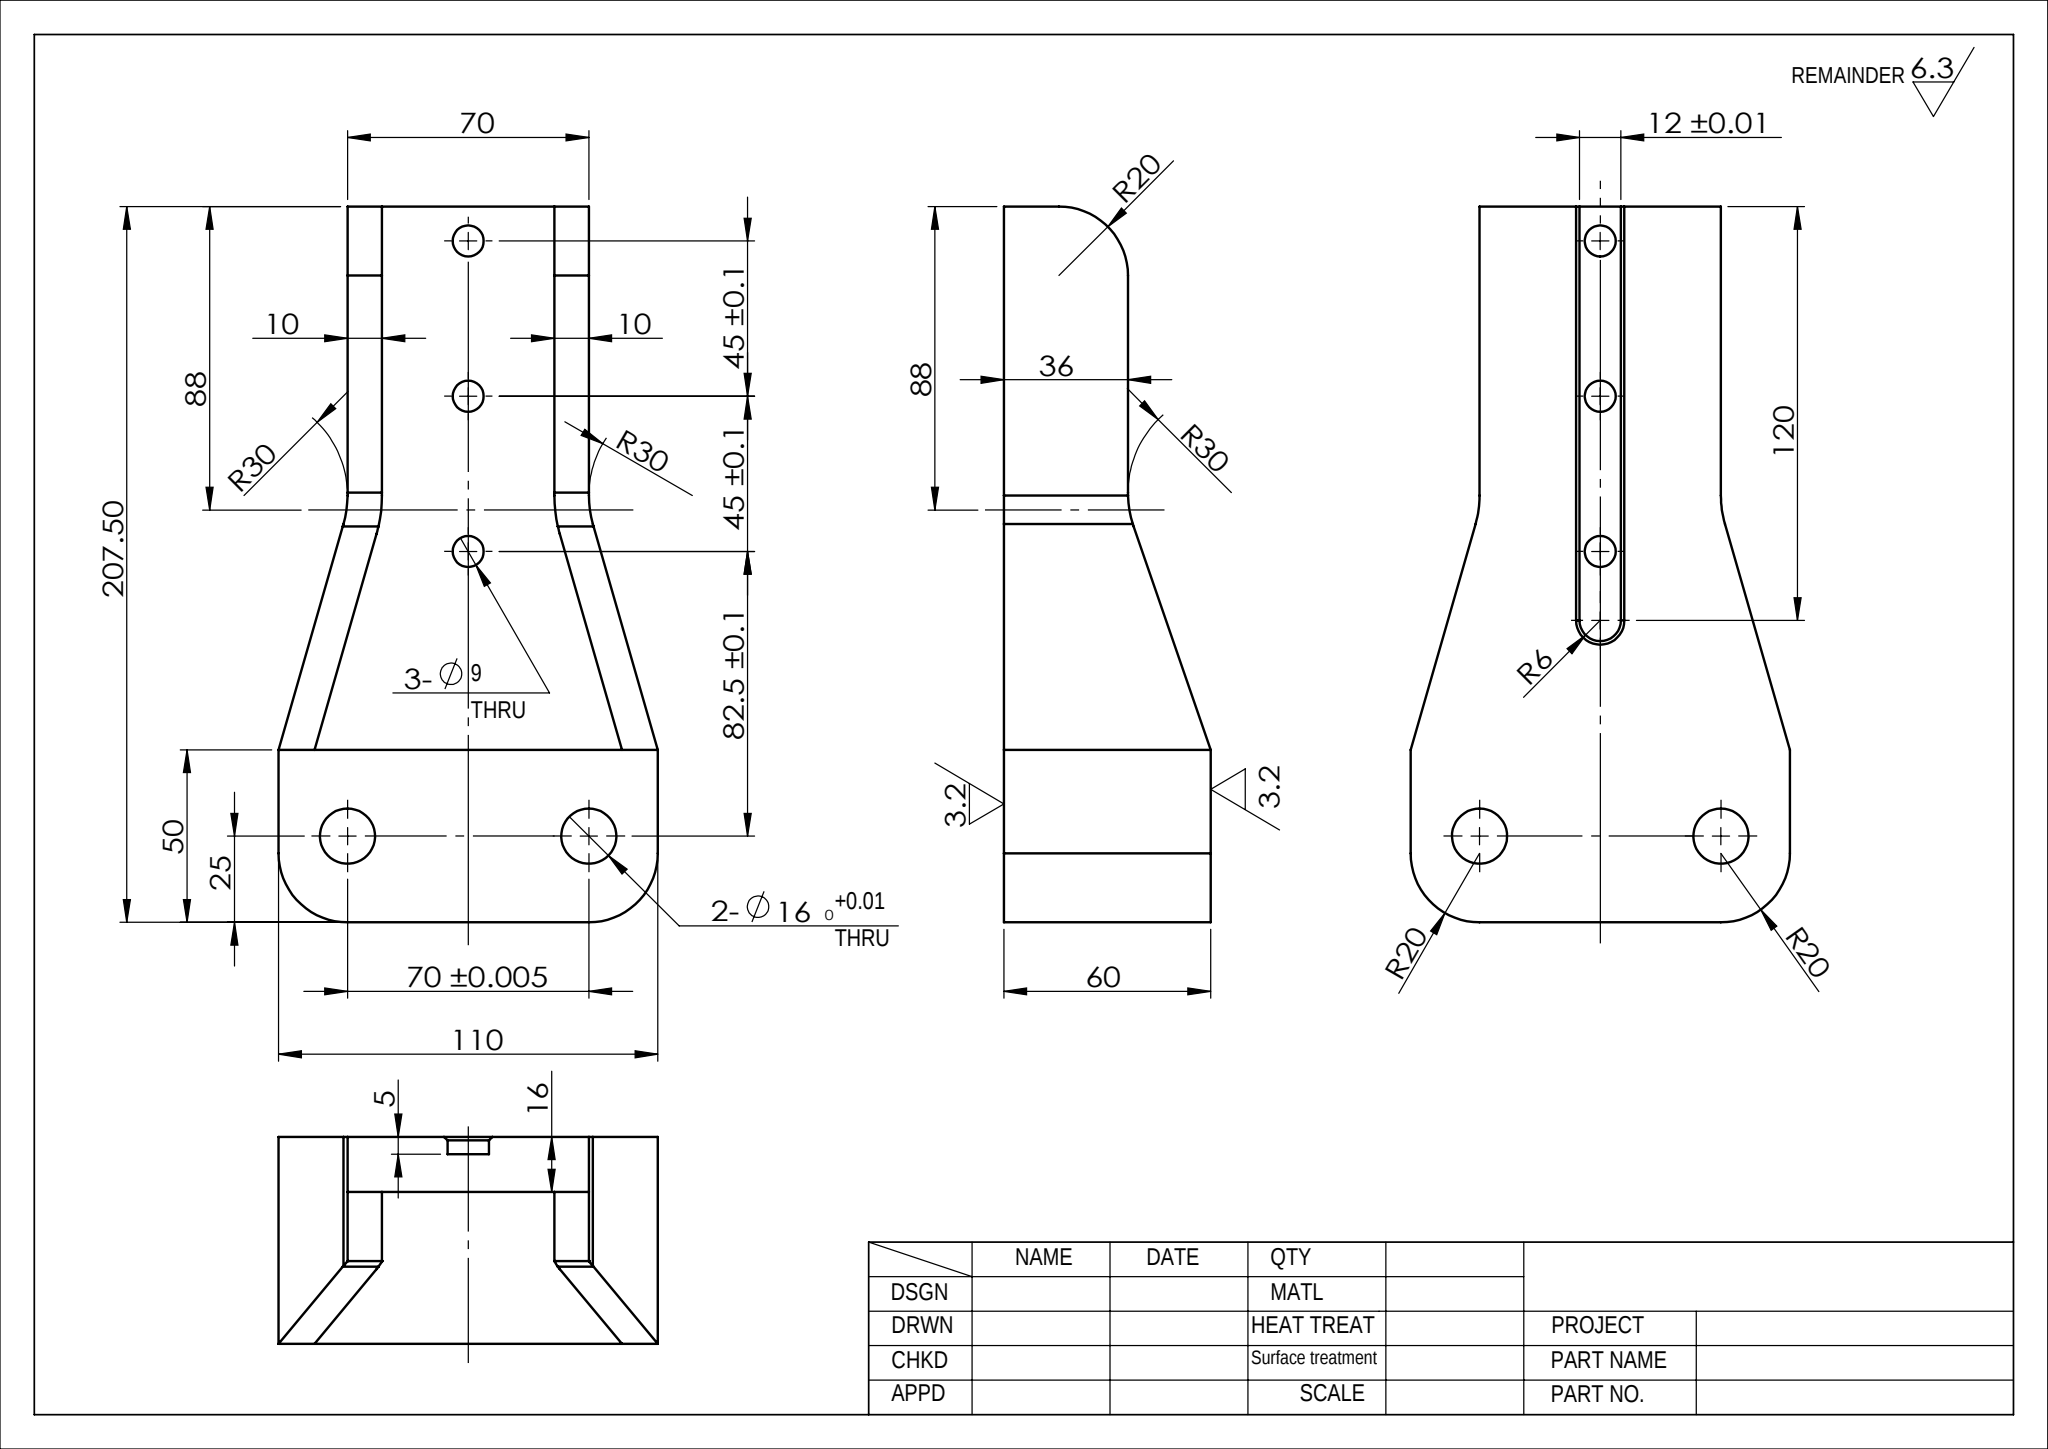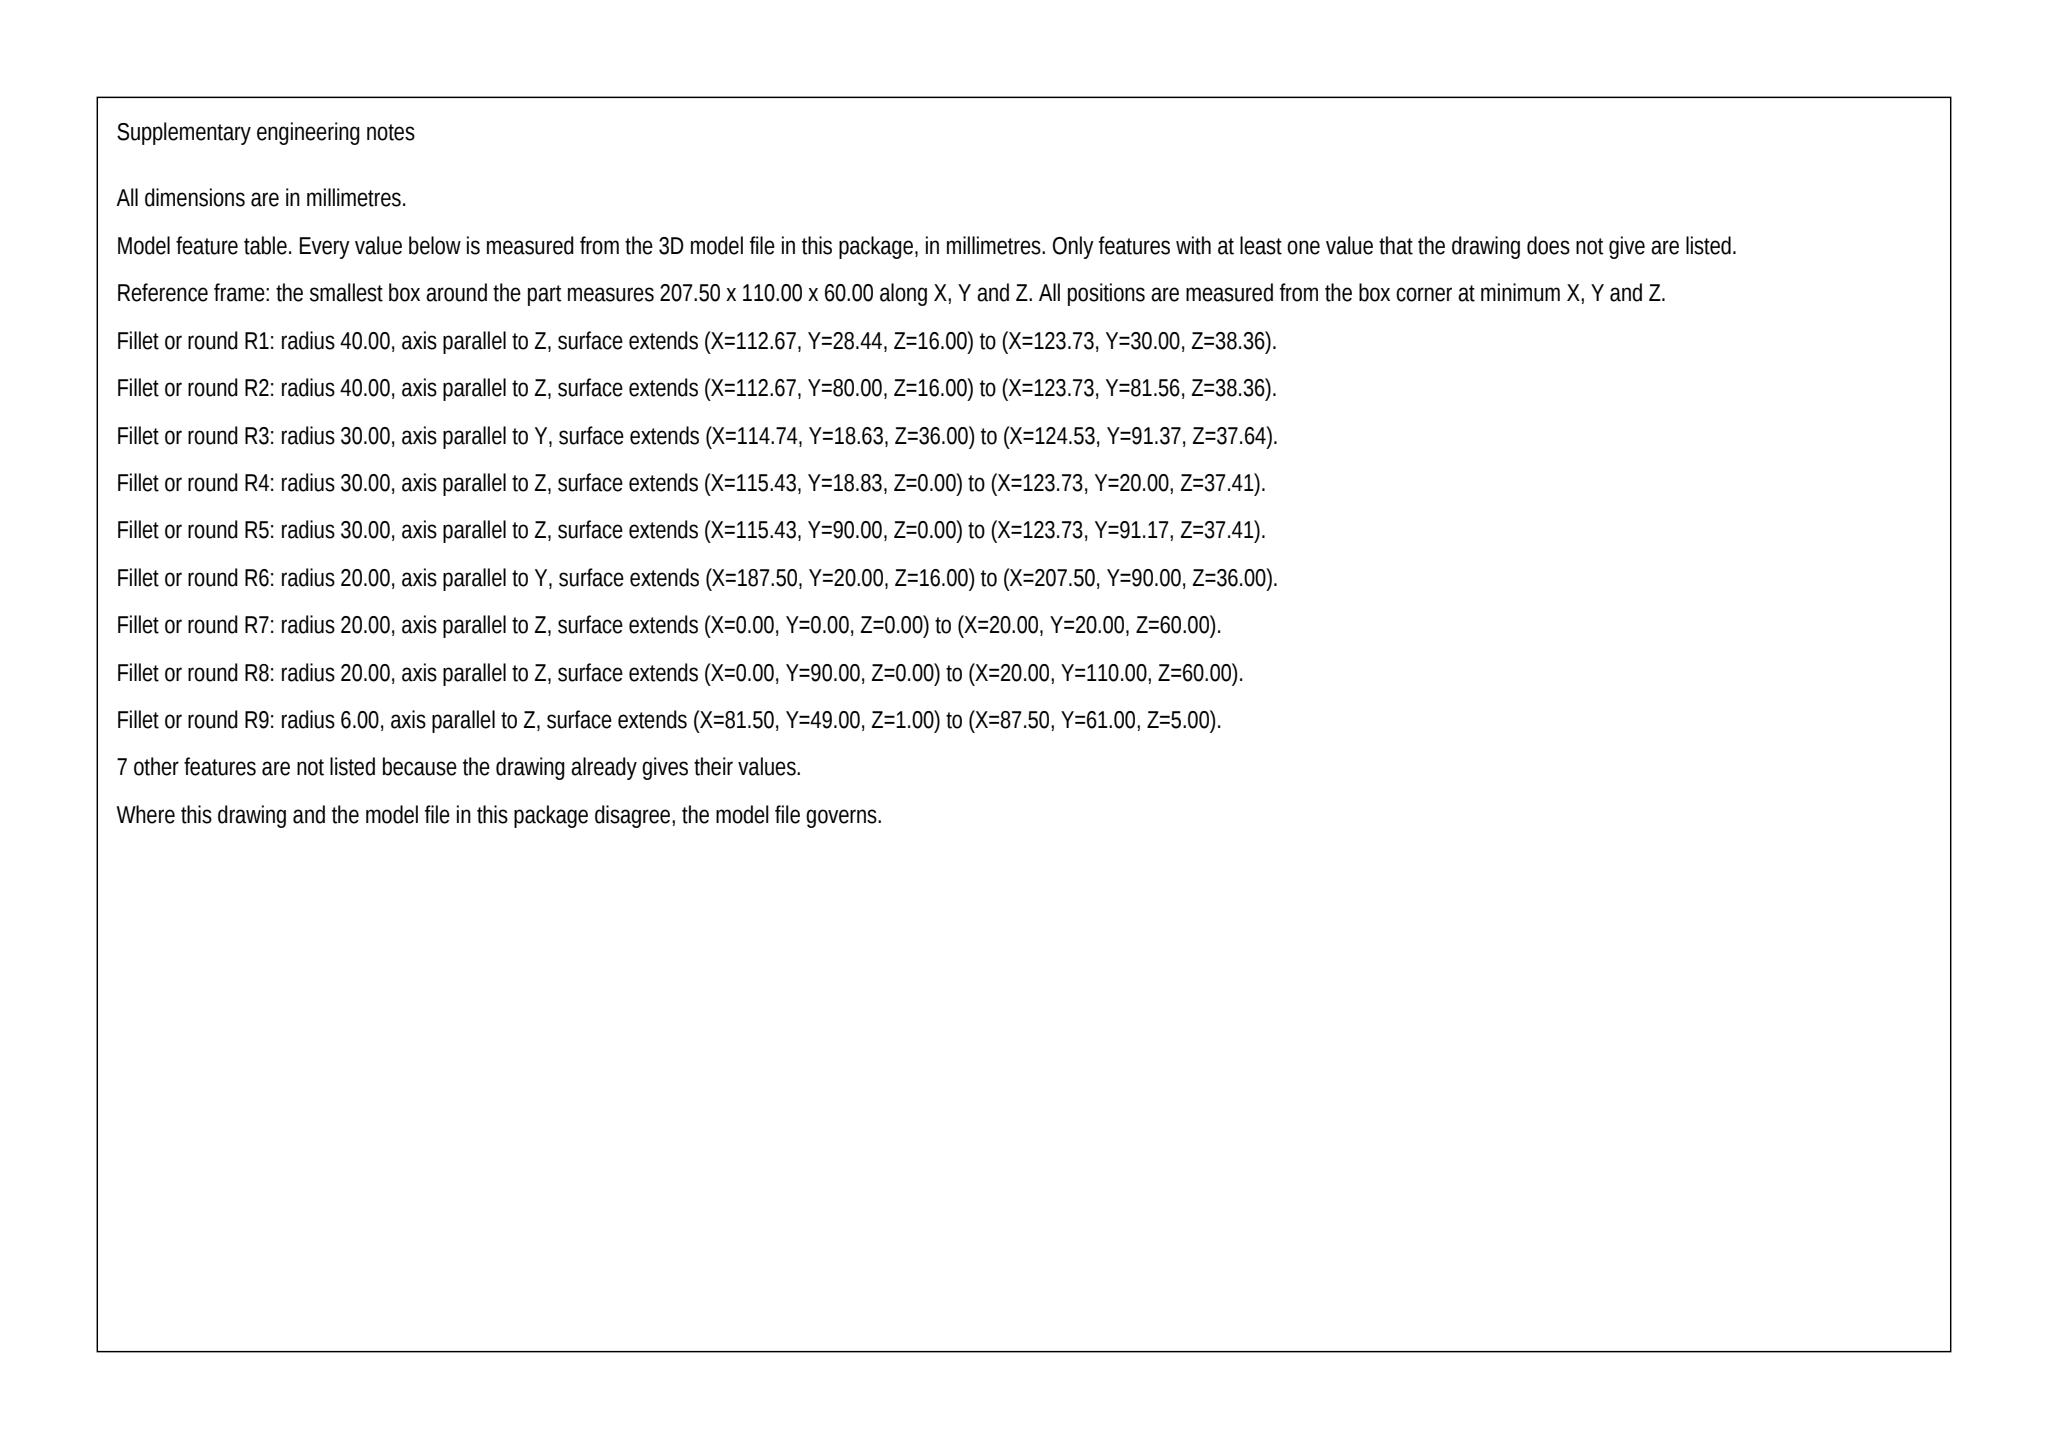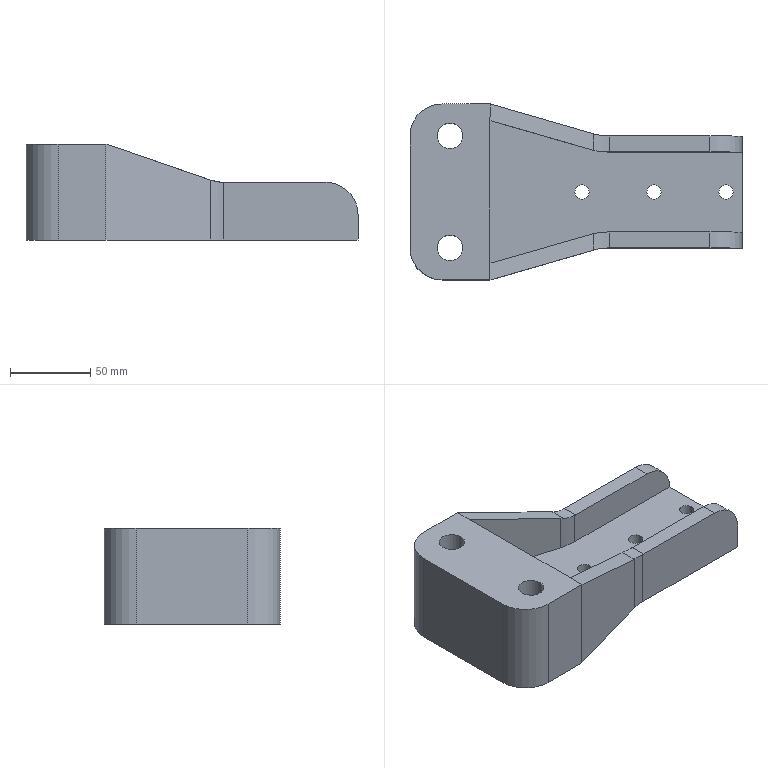Part | SolidWorks | mm | 1 solid | 49 faces | box 207.5 x 110 x 60 mm | volume 564284 mm3 | plane 25 | cylinder 22 | cone 2 | commonest cylinder face diameters 9 x6 16 x4 40 x4 60 x4 12 x2 80 x2
build123d program:
from build123d import *

# Parameters (mm, degrees)
SKETCH1_W          = 50
SKETCH1_H          = 110
SKETCH1_R          = 8
EXTRUDE1_DEPTH     = 60
FILLET1_R          = 20
SKETCH2_W          = 16
SKETCH2_H          = 110
EXTRUDE2_DEPTH     = 157.5
CUT_EXTRUDE1_DEPTH = 213.147
EXTRUDE3_DEPTH     = 44
CUT_EXTRUDE2_DEPTH = 100
FILLET2_R          = 20
CUT_EXTRUDE3_DEPTH = 5
SKETCH7_R          = 4.5
CUT_EXTRUDE4_DEPTH = 211.787
CHAMFER1_SIZE      = 1
FILLET5_R          = 30


with BuildPart() as part:
    # Sketch1 → Extrude1 (new body)
    with BuildSketch(Plane.XY):
        with Locations((0, 35)):
            Rectangle(SKETCH1_W, SKETCH1_H)
        Circle(SKETCH1_R, mode=Mode.SUBTRACT)
        with Locations((0, 70)):
            Circle(SKETCH1_R, mode=Mode.SUBTRACT)
    extrude(amount=EXTRUDE1_DEPTH)

    # Fillet1
    fillet1_edges = [part.edges().sort_by_distance(p)[0] for p in [
        (-25, 90, 30),
        (-25, -20, 30),
    ]]
    fillet(fillet1_edges, radius=FILLET1_R)

    # Sketch2 → Extrude2 (add)
    with BuildSketch(Plane(origin=(25, 0, 0), x_dir=(0, 0, -1), z_dir=(1, 0, 0))):
        with Locations((-8, 35)):
            Rectangle(SKETCH2_W, SKETCH2_H)
    extrude(amount=EXTRUDE2_DEPTH)

    # Sketch3 → Cut-Extrude1 (cut, through all)
    with BuildSketch(Plane(origin=(0, 0, 0), x_dir=(-1, 0, 0), z_dir=(0, 0, -1))):
        with BuildLine():
            Line((-90.434, 71.17), (-25, 90))
            Line((-25, 90), (-182.5, 90))
            Line((-182.5, 90), (-182.5, 70))
            Line((-182.5, 70), (-98.731, 70))
            ThreePointArc((-98.731, 70), (-94.541, 70.294), (-90.434, 71.17))
        make_face()
        with BuildLine():
            Line((-182.5, 0), (-98.731, 0))
            ThreePointArc((-98.731, 0), (-94.541, -0.2939), (-90.434, -1.17))
            Line((-90.434, -1.17), (-25, -20))
            Line((-25, -20), (-182.5, -20))
            Line((-182.5, -20), (-182.5, 0))
        make_face()
    extrude(amount=-CUT_EXTRUDE1_DEPTH, mode=Mode.SUBTRACT)

    # Sketch4 → Extrude3 (add)
    with BuildSketch(Plane.XY.offset(16)):
        with BuildLine():
            Line((25, -9.594), (87.669, 8.44))
            ThreePointArc((87.669, 8.44), (93.145, 9.608), (98.731, 10))
            Line((98.731, 10), (182.5, 10))
            Line((182.5, 10), (182.5, 0))
            Line((182.5, 0), (98.731, 0))
            ThreePointArc((98.731, 0), (94.541, -0.2939), (90.434, -1.17))
            Line((90.434, -1.17), (25, -20))
            Line((25, -20), (25, -9.594))
        make_face()
        with BuildLine():
            Line((182.5, 70), (98.731, 70))
            ThreePointArc((98.731, 70), (94.541, 70.294), (90.434, 71.17))
            Line((90.434, 71.17), (25, 90))
            Line((25, 90), (25, 79.594))
            Line((25, 79.594), (87.669, 61.56))
            ThreePointArc((87.669, 61.56), (93.145, 60.392), (98.731, 60))
            Line((98.731, 60), (182.5, 60))
            Line((182.5, 60), (182.5, 70))
        make_face()
    extrude(amount=EXTRUDE3_DEPTH)

    # Sketch5 → Cut-Extrude2 (cut, symmetric)
    with BuildSketch(Plane.XZ):
        Polygon((25, 60), (94.5, 36), (182.5, 36), (182.5, 60), align=None)
    extrude(amount=CUT_EXTRUDE2_DEPTH, both=True, mode=Mode.SUBTRACT)

    # Fillet2
    fillet2_edges = [part.edges().sort_by_distance(p)[0] for p in [
        (182.5, 65, 36),
        (182.5, 5, 36),
    ]]
    fillet(fillet2_edges, radius=FILLET2_R)

    # Sketch6 → Cut-Extrude3 (cut)
    with BuildSketch(Plane(origin=(0, 0, 0), x_dir=(-1, 0, 0), z_dir=(0, 0, -1))):
        with BuildLine():
            Line((-253.571, 29), (-62.5, 29))
            ThreePointArc((-62.5, 29), (-56.5, 35), (-62.5, 41))
            Line((-62.5, 41), (-253.571, 41))
            Line((-253.571, 41), (-253.571, 29))
        make_face()
    extrude(amount=-CUT_EXTRUDE3_DEPTH, mode=Mode.SUBTRACT)

    # Sketch7 → Cut-Extrude4 (cut, through all)
    with BuildSketch(Plane(origin=(0, 0, 5), x_dir=(-1, 0, 0), z_dir=(0, 0, -1))):
        with Locations((-172.5, 35)):
            Circle(SKETCH7_R)
        with Locations((-127.5, 35)):
            Circle(SKETCH7_R)
        with Locations((-82.5, 35)):
            Circle(SKETCH7_R)
    extrude(amount=-CUT_EXTRUDE4_DEPTH, mode=Mode.SUBTRACT)

    # Chamfer1
    chamfer1_edges = [part.edges().sort_by_distance(p)[0] for p in [
        (122.5, 41, 0),
        (122.5, 29, 0),
        (56.5, 35, 0),
    ]]
    chamfer(chamfer1_edges, length=CHAMFER1_SIZE)

    # Fillet5
    fillet5_edges = [part.edges().sort_by_distance(p)[0] for p in [
        (94.5, 4.738, 36),
        (94.5, 65.262, 36),
    ]]
    fillet(fillet5_edges, radius=FILLET5_R)


solid = part.part